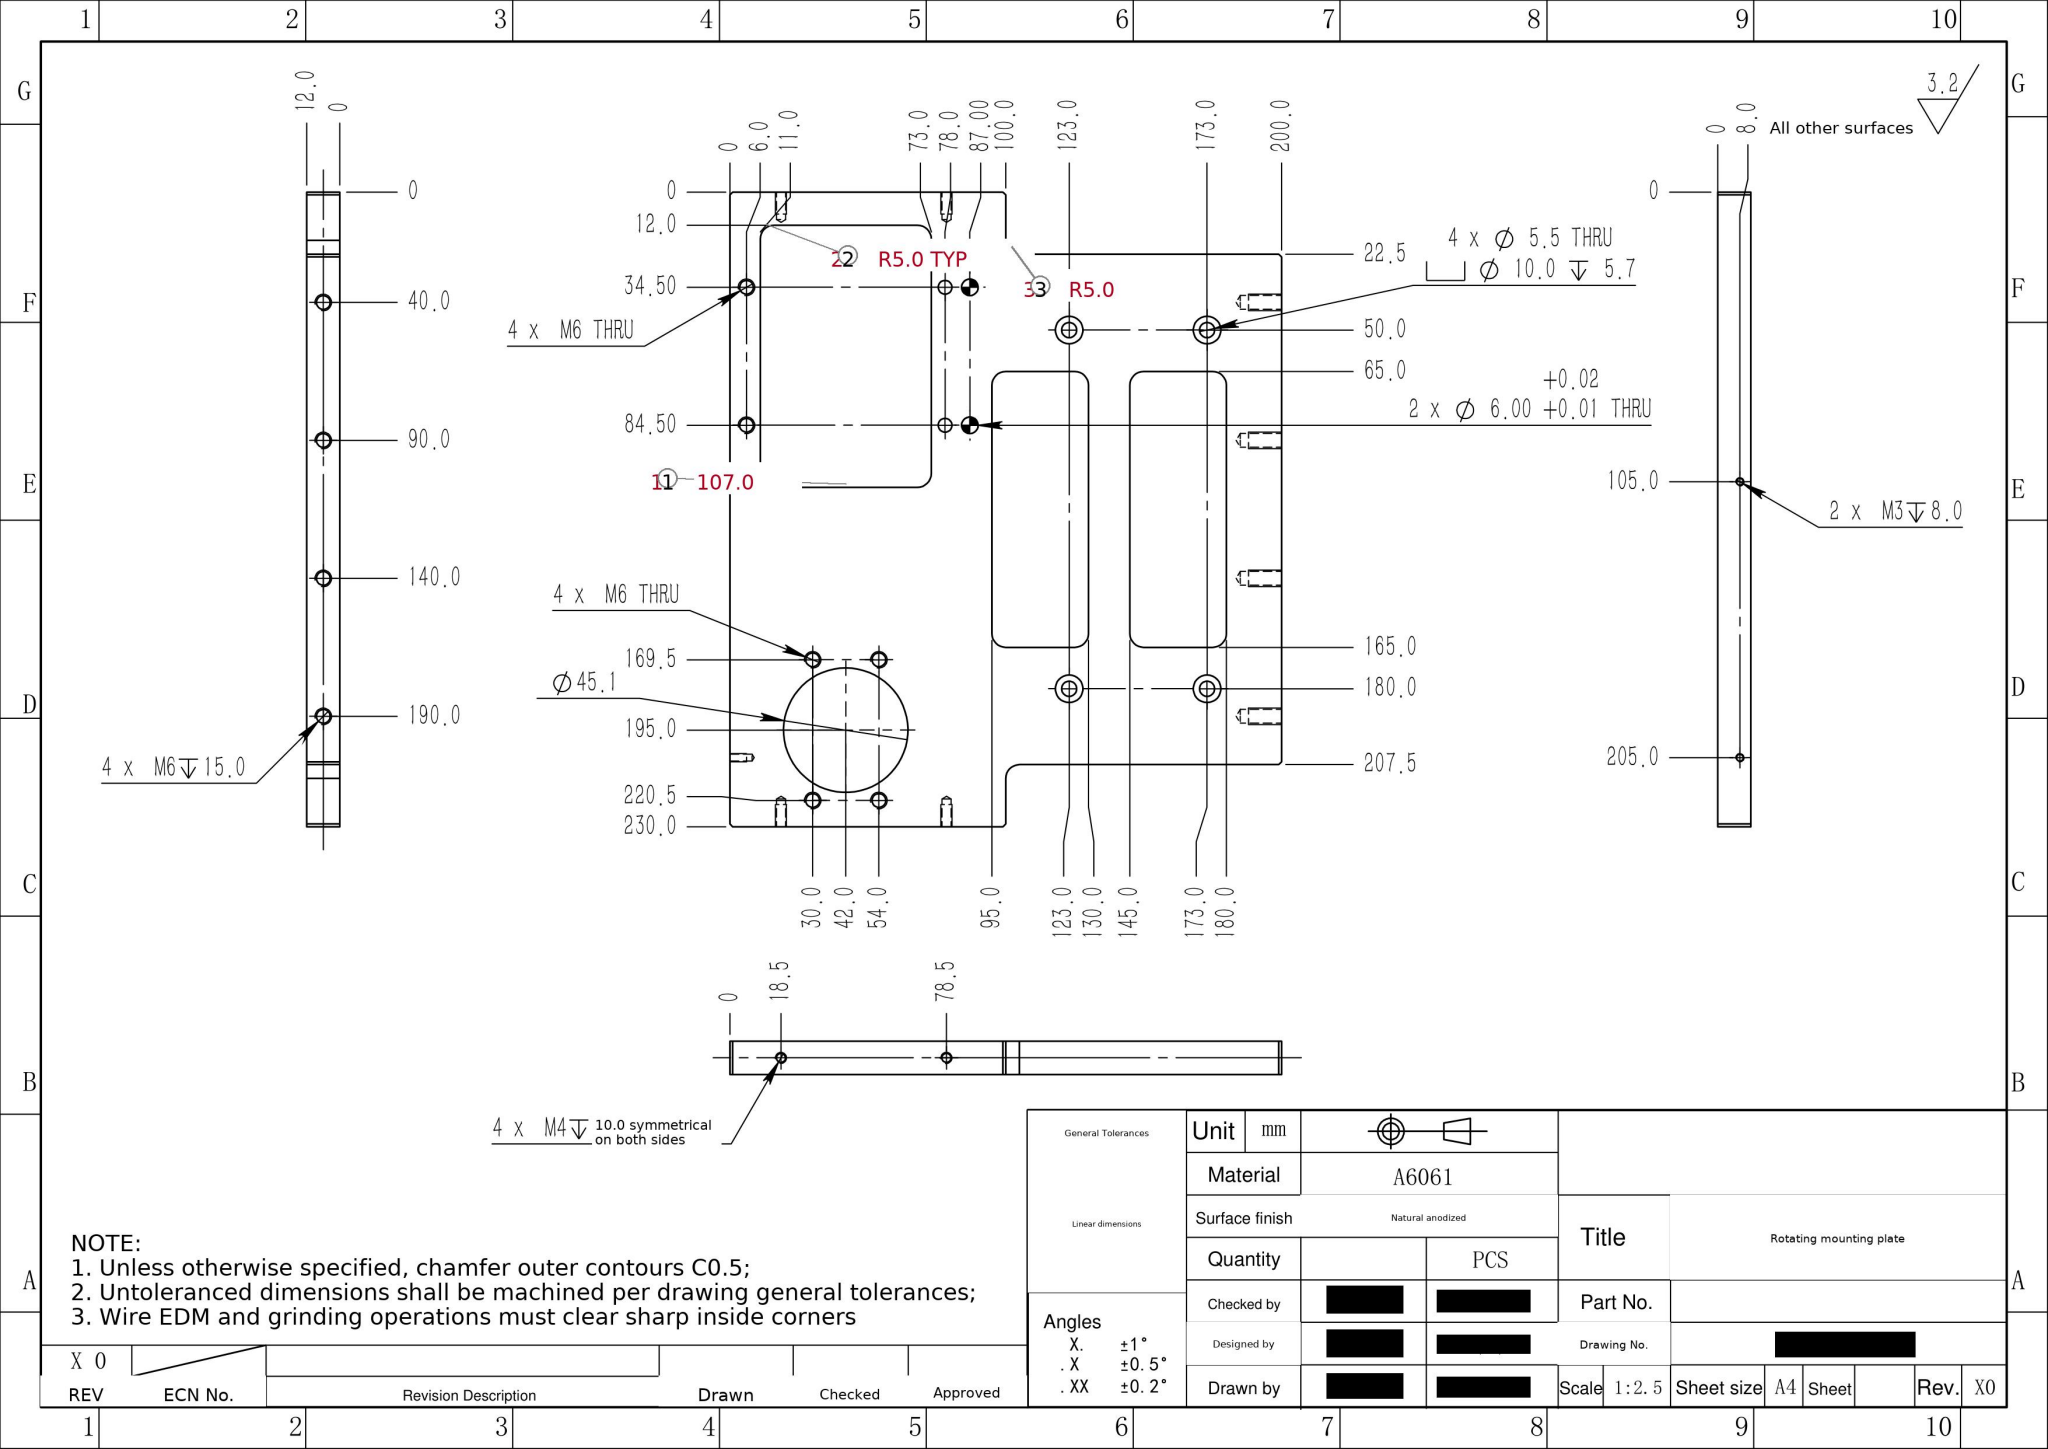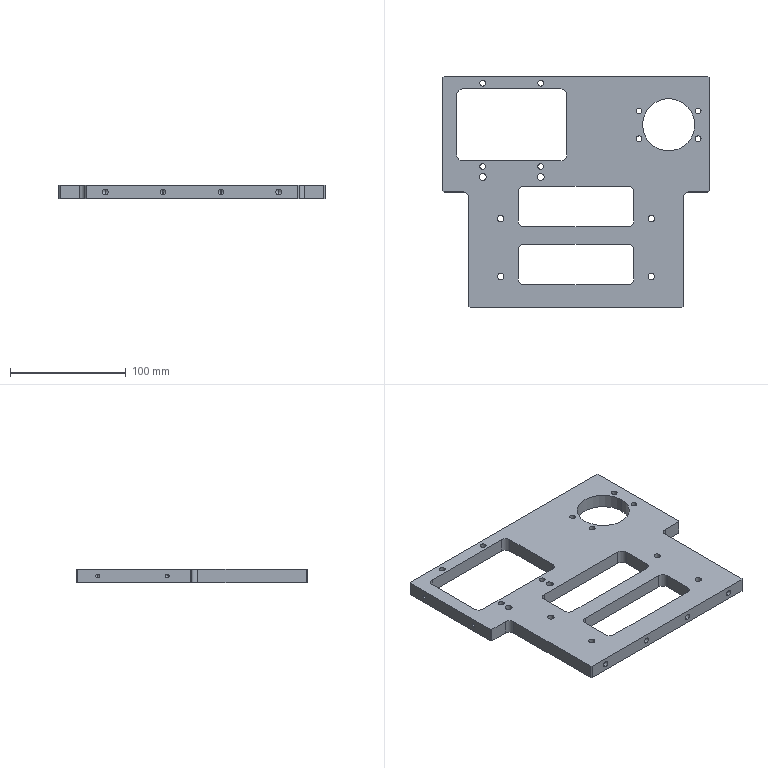Part | SolidWorks | mm | material A6061 | 1 solid | 124 faces | box 230 x 200 x 12 mm | volume 318410 mm3 | cylinder 72 | plane 32 | cone 20 | commonest cylinder face diameters 5 x24 10 x22 3.3 x8 5.5 x8 2.5 x4 6 x4 45.1 x2
build123d program:
from build123d import *

# Parameters (mm, degrees)
SKETCH1_W                                          = 230
SKETCH1_H                                          = 200
BOSS_EXTRUDE1_DEPTH                                = 6
SKETCH9_R                                          = 22.55
CUT_EXTRUDE2_DEPTH                                 = 153.869
M6_TAPPED_HOLE1_D                                  = 5
SKETCH18_W                                         = 95
SKETCH18_H                                         = 62
CUT_EXTRUDE4_DEPTH                                 = 153.869
M6_TAPPED_HOLE3_D                                  = 5
M6_TAPPED_HOLE2_D                                  = 5
M6_TAPPED_HOLE2_DEPTH                              = 15
M6_TAPPED_HOLE2_TIP                                = 1.502
HOLE_SIZE_ACCORDING_TO_TYPE_1_OF_HEXAG_D           = 5.5
HOLE_SIZE_ACCORDING_TO_TYPE_1_OF_HEXAG_CBORE_D     = 10
HOLE_SIZE_ACCORDING_TO_TYPE_1_OF_HEXAG_CBORE_DEPTH = 5.7
SKETCH36_W                                         = 22.5
SKETCH36_H                                         = 100
CUT_EXTRUDE5_DEPTH                                 = 153.869
SKETCH37_W                                         = 100
SKETCH37_H                                         = 35
CUT_EXTRUDE6_DEPTH                                 = 153.869
SIZE_MM_DOWEL_PIN_HOLE_1_D                         = 6
M3_TAPPED_HOLE2_D                                  = 2.5
M3_TAPPED_HOLE2_DEPTH                              = 8
M3_TAPPED_HOLE2_TIP                                = 0.7511
M4_TAPPED_HOLE1_AT_2_COUNT                         = 2
M4_TAPPED_HOLE1_AT_2_PITCH                         = 60
FILLET1_R                                          = 5
CHAMFER1_SIZE                                      = 1


with BuildPart() as part:
    # Sketch1 → Boss-Extrude1 (new, symmetric)
    with BuildSketch(Plane.XY):
        Rectangle(SKETCH1_W, SKETCH1_H)
    extrude(amount=BOSS_EXTRUDE1_DEPTH, both=True)

    # Sketch9 → Cut-Extrude2 (cut, through all)
    with BuildSketch(Plane(origin=(0, 0, -6), x_dir=(-1, 0, 0), z_dir=(0, 0, -1))):
        with Locations((-80, 58)):
            Circle(SKETCH9_R)
    extrude(amount=-CUT_EXTRUDE2_DEPTH, mode=Mode.SUBTRACT)

    # M6 Tapped Hole1 (through all)
    with Locations(Plane(origin=(0, 0, -6), x_dir=(-1, 0, 0), z_dir=(0, 0, -1))):
        with Locations((-105.5, 70), (-54.5, 46), (-54.5, 70), (-105.5, 46)):
            Hole(M6_TAPPED_HOLE1_D / 2)

    # Sketch18 → Cut-Extrude4 (cut, through all)
    with BuildSketch(Plane.XY.offset(6)):
        with Locations((-55.5, 58)):
            Rectangle(SKETCH18_W, SKETCH18_H)
    extrude(amount=-CUT_EXTRUDE4_DEPTH, mode=Mode.SUBTRACT)

    # M6 Tapped Hole3 (through all)
    with Locations(Plane(origin=(0, 0, -6), x_dir=(1, 0, 0), z_dir=(0, 0, -1))):
        with Locations((-30.5, -22), (-30.5, -94), (-80.5, -94), (-80.5, -22)):
            Hole(M6_TAPPED_HOLE3_D / 2)

    # M6 Tapped Hole2
    with Locations(Plane(origin=(0, -100, 0), x_dir=(-1, 0, 0), z_dir=(0, -1, 0))):
        with Locations((25, 0), (-25, 0), (-75, 0), (75, 0)):
            Hole(M6_TAPPED_HOLE2_D / 2, depth=M6_TAPPED_HOLE2_DEPTH)
            with Locations((0, 0, -(M6_TAPPED_HOLE2_DEPTH + M6_TAPPED_HOLE2_TIP / 2))):  # 118° drill point
                Cone(0, M6_TAPPED_HOLE2_D / 2, M6_TAPPED_HOLE2_TIP, mode=Mode.SUBTRACT)

    # Hole Size _According to_ Type 1 of Hexag (through all)
    with Locations(Plane(origin=(0, 0, -6), x_dir=(-1, 0, 0), z_dir=(0, 0, -1))):
        with Locations((-65, -23), (-65, -73), (65, -73), (65, -23)):
            CounterBoreHole(HOLE_SIZE_ACCORDING_TO_TYPE_1_OF_HEXAG_D / 2, HOLE_SIZE_ACCORDING_TO_TYPE_1_OF_HEXAG_CBORE_D / 2, HOLE_SIZE_ACCORDING_TO_TYPE_1_OF_HEXAG_CBORE_DEPTH)

    # Sketch36 → Cut-Extrude5 (cut, through all)
    with BuildSketch(Plane(origin=(0, 0, -6), x_dir=(-1, 0, 0), z_dir=(0, 0, -1))):
        with Locations((-103.75, -50)):
            Rectangle(SKETCH36_W, SKETCH36_H)
        with Locations((103.75, -50)):
            Rectangle(SKETCH36_W, SKETCH36_H)
    extrude(amount=-CUT_EXTRUDE5_DEPTH, mode=Mode.SUBTRACT)

    # Sketch37 → Cut-Extrude6 (cut, through all)
    with BuildSketch(Plane.XY.offset(6)):
        with Locations((0, -12.5)):
            Rectangle(SKETCH37_W, SKETCH37_H)
        with Locations((0, -62.5)):
            Rectangle(SKETCH37_W, SKETCH37_H)
    extrude(amount=-CUT_EXTRUDE6_DEPTH, mode=Mode.SUBTRACT)

    # Size mm Dowel Pin Hole 1 (through all)
    with Locations(Plane.XY.offset(6)):
        with Locations((-80.5, 13), (-30.5, 13)):
            Hole(SIZE_MM_DOWEL_PIN_HOLE_1_D / 2)

    # M3 Tapped Hole2
    with Locations(Plane(origin=(0, 100, 0), x_dir=(1, 0, 0), z_dir=(0, 1, 0))):
        with Locations((90, 2), (-10, 2)):
            Hole(M3_TAPPED_HOLE2_D / 2, depth=M3_TAPPED_HOLE2_DEPTH)
            with Locations((0, 0, -(M3_TAPPED_HOLE2_DEPTH + M3_TAPPED_HOLE2_TIP / 2))):  # 118° drill point
                Cone(0, M3_TAPPED_HOLE2_D / 2, M3_TAPPED_HOLE2_TIP, mode=Mode.SUBTRACT)

    # Sketch43 → M4 Tapped Hole1 (revolve, cut)
    with BuildSketch(Plane(origin=(-115, 81.5, 0), x_dir=(0, 0, 1), z_dir=(0, 1, 0))):
        Polygon((0, 0), (0, 10.991), (1.65, 10), (1.65, 0), align=None)
    m4_tapped_hole1 = revolve(axis=Axis((-121.35, 81.5, 0), (1, 0, 0)), mode=Mode.SUBTRACT)

    # M4 Tapped Hole1 at 2: M4 Tapped Hole1 ×2
    with Locations(*[(0, -i * M4_TAPPED_HOLE1_AT_2_PITCH, 0) for i in range(1, M4_TAPPED_HOLE1_AT_2_COUNT)]):
        add(m4_tapped_hole1, mode=Mode.SUBTRACT)

    # Mirror1: M4 Tapped Hole1 across plane
    add(m4_tapped_hole1.mirror(Plane(origin=(0, 0, 0), x_dir=(0, 0, 1), z_dir=(1, 0, 0))), mode=Mode.SUBTRACT)

    # Mirror1 copy 1 sketch → Mirror1 copy 1 (revolve, cut)
    with BuildSketch(Plane(origin=(115, 21.5, 0), x_dir=(0, 0, 1), z_dir=(0, 1, 0))):
        Polygon((0, 0), (0, -10.991), (1.65, -10), (1.65, 0), align=None)
    revolve(axis=Axis((121.35, 21.5, 0), (1, 0, 0)), mode=Mode.SUBTRACT)

    # Fillet1
    fillet1_edges = [part.edges().sort_by_distance(p)[0] for p in [
        (92.5, 0, 0),
        (-92.5, 0, 0),
        (-50, -30, 0),
        (-50, 5, 0),
        (50, 5, 0),
        (50, -30, 0),
        (-50, -80, 0),
        (-50, -45, 0),
        (50, -45, 0),
        (50, -80, 0),
        (-8, 89, 0),
        (-8, 27, 0),
        (-103, 27, 0),
        (-103, 89, 0),
    ]]
    fillet(fillet1_edges, radius=FILLET1_R)

    # Chamfer1
    chamfer1_edges = [part.edges().sort_by_distance(p)[0] for p in [
        (115, 0, 0),
        (92.5, -100, 0),
        (-115, 0, 0),
        (-92.5, -100, 0),
        (-115, 100, 0),
        (115, 100, 0),
    ]]
    chamfer(chamfer1_edges, length=CHAMFER1_SIZE)


solid = part.part